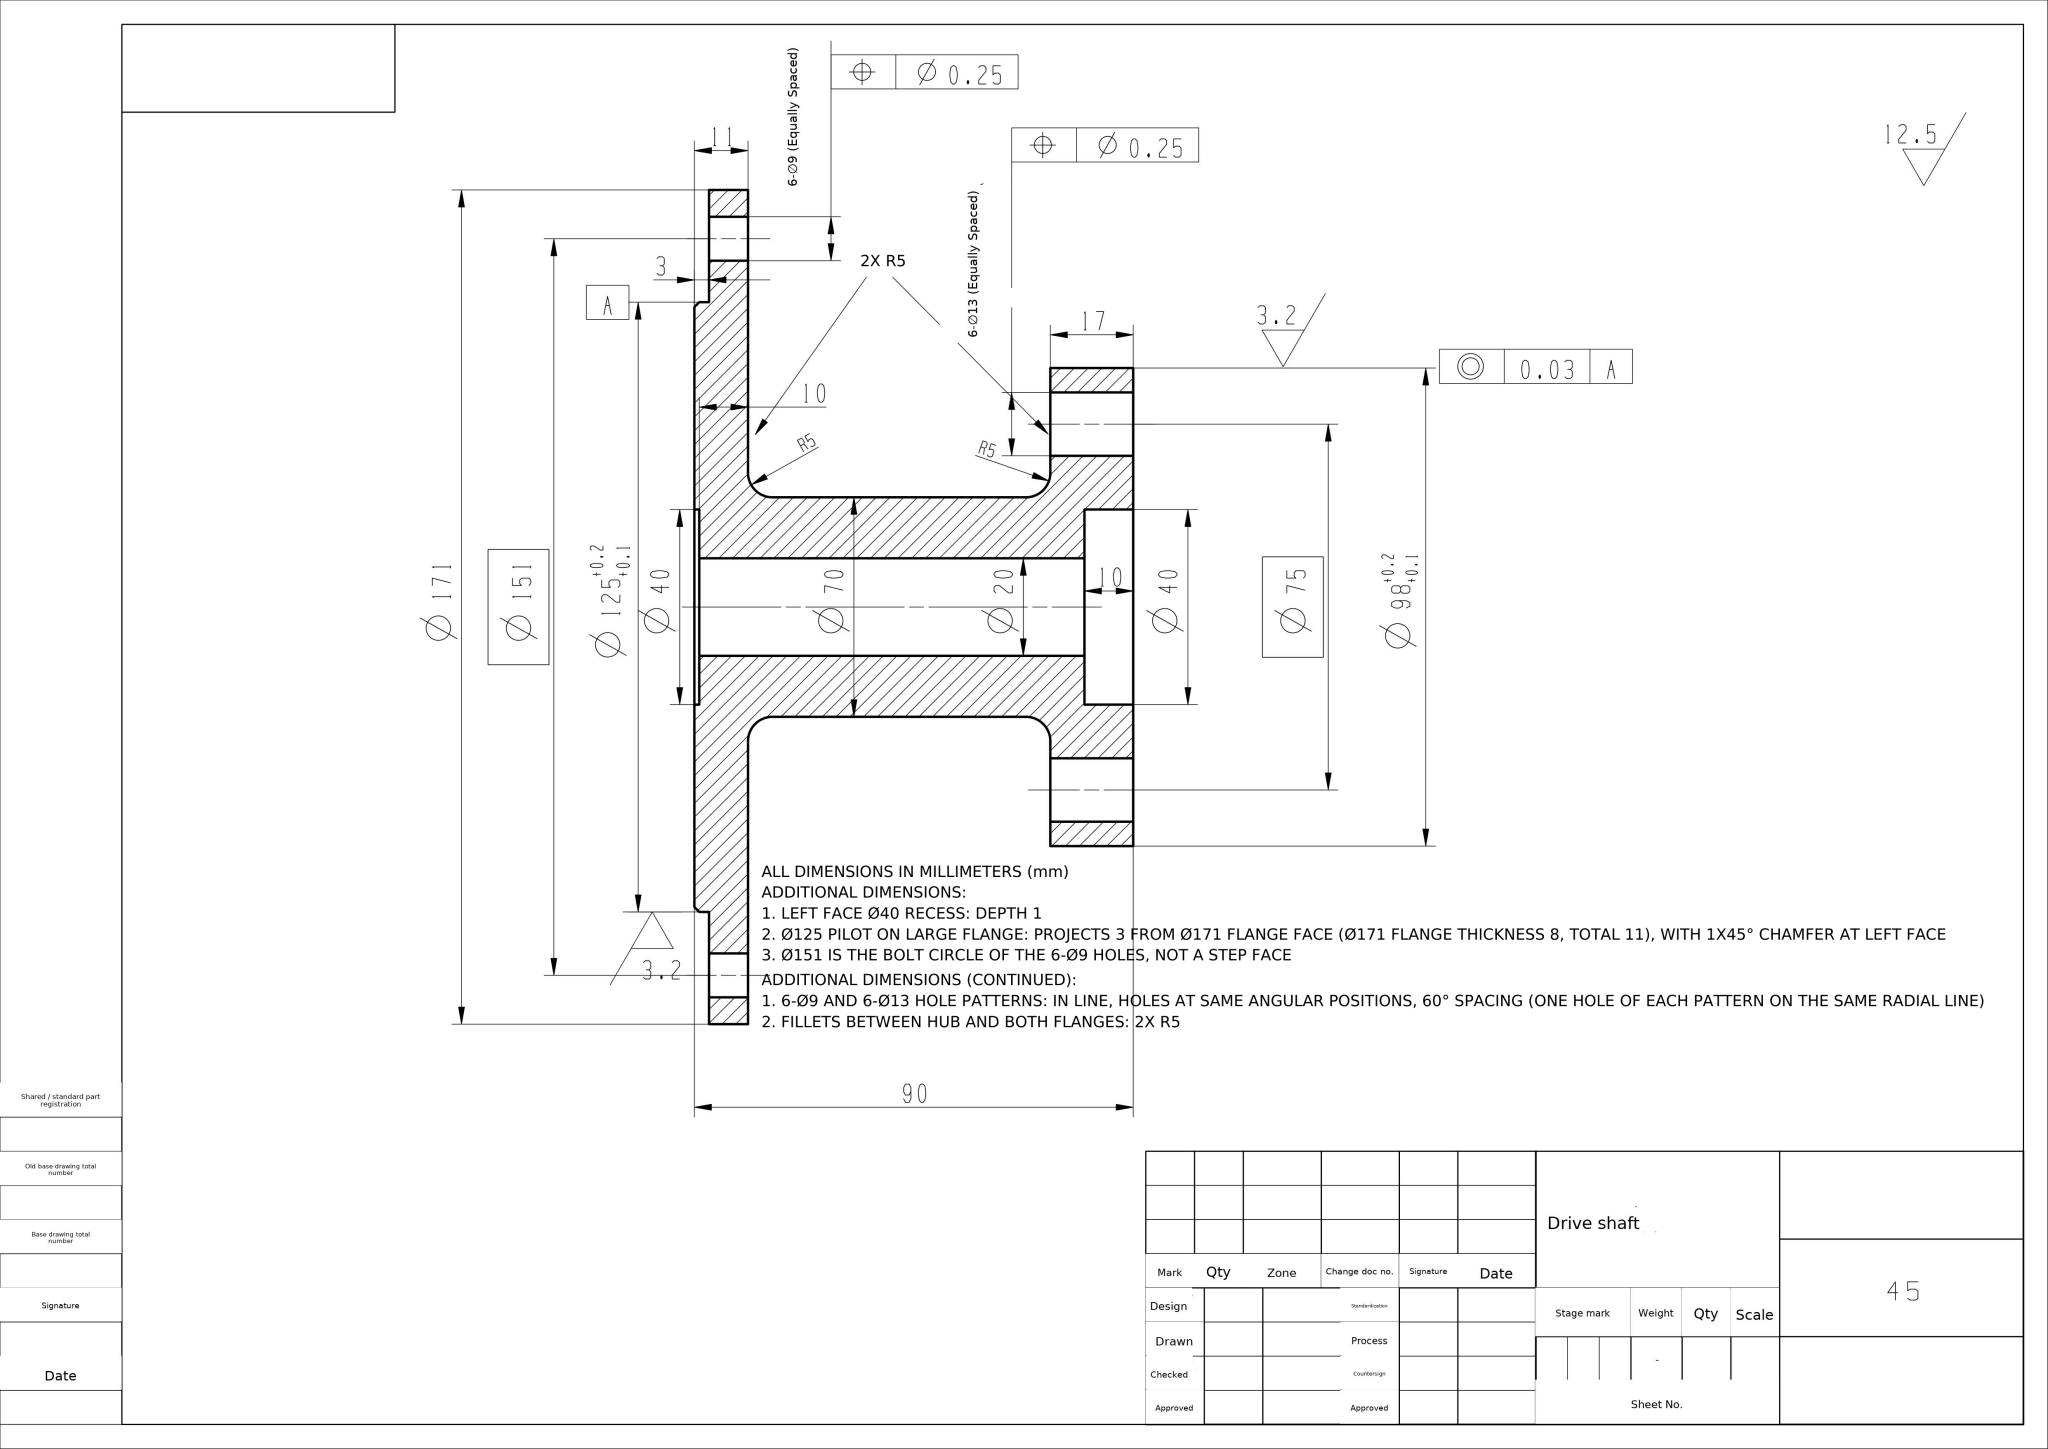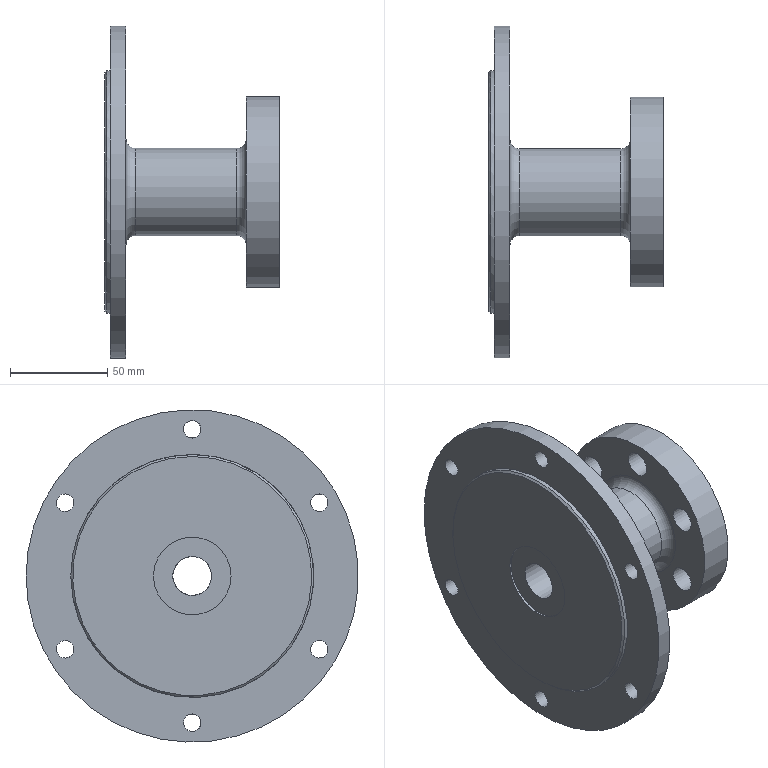Part | NX | mm | 1 solid | 29 faces | box 90 x 171 x 171 mm | volume 393542 mm3 | cylinder 19 | plane 7 | torus 2 | cone 1 | commonest cylinder face diameters 13 x6 9 x6 40 x2 45 x1 98 x1 171 x1 125 x1 20 x1
STEP:
#1=CARTESIAN_POINT('',(0.,0.,0.));
#2=DIRECTION('',(0.,0.,1.));
#3=DIRECTION('',(1.,0.,0.));
#4=AXIS2_PLACEMENT_3D('',#1,#2,#3);
#5=(LENGTH_UNIT()NAMED_UNIT(*)SI_UNIT(.MILLI.,.METRE.));
#6=UNCERTAINTY_MEASURE_WITH_UNIT(LENGTH_MEASURE(0.00002),#5,'','');
#7=(NAMED_UNIT(*)PLANE_ANGLE_UNIT()SI_UNIT($,.RADIAN.));
#8=PLANE_ANGLE_MEASURE_WITH_UNIT(PLANE_ANGLE_MEASURE(0.01745),#7);
#9=DIMENSIONAL_EXPONENTS(0.,0.,0.,0.,0.,0.,0.);
#10=(CONVERSION_BASED_UNIT('',#8)NAMED_UNIT(#9)PLANE_ANGLE_UNIT());
#11=(NAMED_UNIT(*)SI_UNIT($,.STERADIAN.)SOLID_ANGLE_UNIT());
#12=(GEOMETRIC_REPRESENTATION_CONTEXT(3)GLOBAL_UNCERTAINTY_ASSIGNED_CONTEXT((#6))GLOBAL_UNIT_ASSIGNED_CONTEXT((#5,#10,#11))REPRESENTATION_CONTEXT('',''));
#13=SHAPE_REPRESENTATION('',(#4),#12);
#14=CARTESIAN_POINT('',(-57.,0.,22.5));
#15=VERTEX_POINT('',#14);
#16=CARTESIAN_POINT('',(-57.,0.,0.));
#17=DIRECTION('',(1.,0.,0.));
#18=DIRECTION('',(0.,0.,1.));
#19=AXIS2_PLACEMENT_3D('',#16,#17,#18);
#20=CIRCLE('',#19,22.5);
#21=EDGE_CURVE('',#15,#15,#20,.T.);
#22=ORIENTED_EDGE('',*,*,#21,.T.);
#23=EDGE_LOOP('',(#22));
#24=FACE_BOUND('',#23,.T.);
#25=CARTESIAN_POINT('',(-5.,0.,-22.5));
#26=VERTEX_POINT('',#25);
#27=CARTESIAN_POINT('',(-5.,0.,0.));
#28=DIRECTION('',(-1.,0.,0.));
#29=DIRECTION('',(0.,0.,-1.));
#30=AXIS2_PLACEMENT_3D('',#27,#28,#29);
#31=CIRCLE('',#30,22.5);
#32=EDGE_CURVE('',#26,#26,#31,.T.);
#33=ORIENTED_EDGE('',*,*,#32,.T.);
#34=EDGE_LOOP('',(#33));
#35=FACE_BOUND('',#34,.T.);
#36=CARTESIAN_POINT('',(-62.,0.,0.));
#37=DIRECTION('',(1.,0.,0.));
#38=DIRECTION('',(0.,0.,-1.));
#39=AXIS2_PLACEMENT_3D('',#36,#37,#38);
#40=CYLINDRICAL_SURFACE('',#39,22.5);
#41=ADVANCED_FACE('',(#24,#35),#40,.T.);
#42=CARTESIAN_POINT('',(17.,0.,-20.));
#43=VERTEX_POINT('',#42);
#44=CARTESIAN_POINT('',(17.,0.,0.));
#45=DIRECTION('',(1.,0.,0.));
#46=DIRECTION('',(0.,0.,-1.));
#47=AXIS2_PLACEMENT_3D('',#44,#45,#46);
#48=CIRCLE('',#47,20.);
#49=EDGE_CURVE('',#43,#43,#48,.T.);
#50=ORIENTED_EDGE('',*,*,#49,.T.);
#51=EDGE_LOOP('',(#50));
#52=FACE_BOUND('',#51,.T.);
#53=CARTESIAN_POINT('',(7.,20.,-0.));
#54=VERTEX_POINT('',#53);
#55=CARTESIAN_POINT('',(7.,0.,0.));
#56=DIRECTION('',(-1.,0.,0.));
#57=DIRECTION('',(0.,1.,-0.));
#58=AXIS2_PLACEMENT_3D('',#55,#56,#57);
#59=CIRCLE('',#58,20.);
#60=EDGE_CURVE('',#54,#54,#59,.T.);
#61=ORIENTED_EDGE('',*,*,#60,.T.);
#62=EDGE_LOOP('',(#61));
#63=FACE_BOUND('',#62,.T.);
#64=CARTESIAN_POINT('',(20.,0.,0.));
#65=DIRECTION('',(-1.,0.,0.));
#66=DIRECTION('',(0.,0.,1.));
#67=AXIS2_PLACEMENT_3D('',#64,#65,#66);
#68=CYLINDRICAL_SURFACE('',#67,20.);
#69=ADVANCED_FACE('',(#52,#63),#68,.F.);
#70=CARTESIAN_POINT('',(17.,49.,-0.));
#71=VERTEX_POINT('',#70);
#72=CARTESIAN_POINT('',(17.,0.,0.));
#73=DIRECTION('',(1.,0.,0.));
#74=DIRECTION('',(0.,1.,-0.));
#75=AXIS2_PLACEMENT_3D('',#72,#73,#74);
#76=CIRCLE('',#75,49.);
#77=EDGE_CURVE('',#71,#71,#76,.T.);
#78=ORIENTED_EDGE('',*,*,#77,.F.);
#79=EDGE_LOOP('',(#78));
#80=FACE_BOUND('',#79,.T.);
#81=CARTESIAN_POINT('',(0.,49.,-0.));
#82=VERTEX_POINT('',#81);
#83=CARTESIAN_POINT('',(0.,0.,0.));
#84=DIRECTION('',(1.,0.,0.));
#85=DIRECTION('',(0.,1.,-0.));
#86=AXIS2_PLACEMENT_3D('',#83,#84,#85);
#87=CIRCLE('',#86,49.);
#88=EDGE_CURVE('',#82,#82,#87,.T.);
#89=ORIENTED_EDGE('',*,*,#88,.T.);
#90=EDGE_LOOP('',(#89));
#91=FACE_BOUND('',#90,.T.);
#92=CARTESIAN_POINT('',(17.,0.,0.));
#93=DIRECTION('',(-1.,0.,0.));
#94=DIRECTION('',(0.,0.,1.));
#95=AXIS2_PLACEMENT_3D('',#92,#93,#94);
#96=CYLINDRICAL_SURFACE('',#95,49.);
#97=ADVANCED_FACE('',(#80,#91),#96,.T.);
#98=CARTESIAN_POINT('',(17.,32.476,12.25));
#99=VERTEX_POINT('',#98);
#100=CARTESIAN_POINT('',(17.,32.476,18.75));
#101=DIRECTION('',(-1.,0.,0.));
#102=DIRECTION('',(0.,0.,-1.));
#103=AXIS2_PLACEMENT_3D('',#100,#101,#102);
#104=CIRCLE('',#103,6.5);
#105=EDGE_CURVE('',#99,#99,#104,.T.);
#106=ORIENTED_EDGE('',*,*,#105,.T.);
#107=EDGE_LOOP('',(#106));
#108=FACE_BOUND('',#107,.T.);
#109=CARTESIAN_POINT('',(17.,32.476,-25.25));
#110=VERTEX_POINT('',#109);
#111=CARTESIAN_POINT('',(17.,32.476,-18.75));
#112=DIRECTION('',(-1.,0.,0.));
#113=DIRECTION('',(0.,0.,-1.));
#114=AXIS2_PLACEMENT_3D('',#111,#112,#113);
#115=CIRCLE('',#114,6.5);
#116=EDGE_CURVE('',#110,#110,#115,.T.);
#117=ORIENTED_EDGE('',*,*,#116,.T.);
#118=EDGE_LOOP('',(#117));
#119=FACE_BOUND('',#118,.T.);
#120=CARTESIAN_POINT('',(17.,-0.,-44.));
#121=VERTEX_POINT('',#120);
#122=CARTESIAN_POINT('',(17.,-0.,-37.5));
#123=DIRECTION('',(-1.,0.,0.));
#124=DIRECTION('',(0.,0.,-1.));
#125=AXIS2_PLACEMENT_3D('',#122,#123,#124);
#126=CIRCLE('',#125,6.5);
#127=EDGE_CURVE('',#121,#121,#126,.T.);
#128=ORIENTED_EDGE('',*,*,#127,.T.);
#129=EDGE_LOOP('',(#128));
#130=FACE_BOUND('',#129,.T.);
#131=CARTESIAN_POINT('',(17.,-32.476,-25.25));
#132=VERTEX_POINT('',#131);
#133=CARTESIAN_POINT('',(17.,-32.476,-18.75));
#134=DIRECTION('',(-1.,0.,0.));
#135=DIRECTION('',(0.,0.,-1.));
#136=AXIS2_PLACEMENT_3D('',#133,#134,#135);
#137=CIRCLE('',#136,6.5);
#138=EDGE_CURVE('',#132,#132,#137,.T.);
#139=ORIENTED_EDGE('',*,*,#138,.T.);
#140=EDGE_LOOP('',(#139));
#141=FACE_BOUND('',#140,.T.);
#142=CARTESIAN_POINT('',(17.,-32.476,12.25));
#143=VERTEX_POINT('',#142);
#144=CARTESIAN_POINT('',(17.,-32.476,18.75));
#145=DIRECTION('',(-1.,0.,0.));
#146=DIRECTION('',(0.,0.,-1.));
#147=AXIS2_PLACEMENT_3D('',#144,#145,#146);
#148=CIRCLE('',#147,6.5);
#149=EDGE_CURVE('',#143,#143,#148,.T.);
#150=ORIENTED_EDGE('',*,*,#149,.T.);
#151=EDGE_LOOP('',(#150));
#152=FACE_BOUND('',#151,.T.);
#153=CARTESIAN_POINT('',(17.,-0.,31.));
#154=VERTEX_POINT('',#153);
#155=CARTESIAN_POINT('',(17.,-0.,37.5));
#156=DIRECTION('',(-1.,0.,0.));
#157=DIRECTION('',(0.,0.,-1.));
#158=AXIS2_PLACEMENT_3D('',#155,#156,#157);
#159=CIRCLE('',#158,6.5);
#160=EDGE_CURVE('',#154,#154,#159,.T.);
#161=ORIENTED_EDGE('',*,*,#160,.T.);
#162=EDGE_LOOP('',(#161));
#163=FACE_BOUND('',#162,.T.);
#164=ORIENTED_EDGE('',*,*,#49,.F.);
#165=EDGE_LOOP('',(#164));
#166=FACE_BOUND('',#165,.T.);
#167=ORIENTED_EDGE('',*,*,#77,.T.);
#168=EDGE_LOOP('',(#167));
#169=FACE_BOUND('',#168,.T.);
#170=CARTESIAN_POINT('',(17.,0.,0.));
#171=DIRECTION('',(1.,0.,0.));
#172=DIRECTION('',(0.,0.,-1.));
#173=AXIS2_PLACEMENT_3D('',#170,#171,#172);
#174=PLANE('',#173);
#175=ADVANCED_FACE('',(#108,#119,#130,#141,#152,#163,#166,#169),#174,.T.);
#176=CARTESIAN_POINT('',(0.,0.,-27.5));
#177=VERTEX_POINT('',#176);
#178=CARTESIAN_POINT('',(0.,0.,0.));
#179=DIRECTION('',(1.,0.,0.));
#180=DIRECTION('',(0.,0.,-1.));
#181=AXIS2_PLACEMENT_3D('',#178,#179,#180);
#182=CIRCLE('',#181,27.5);
#183=EDGE_CURVE('',#177,#177,#182,.T.);
#184=ORIENTED_EDGE('',*,*,#183,.T.);
#185=EDGE_LOOP('',(#184));
#186=FACE_BOUND('',#185,.T.);
#187=CARTESIAN_POINT('',(0.,35.726,13.121));
#188=VERTEX_POINT('',#187);
#189=CARTESIAN_POINT('',(0.,32.476,18.75));
#190=DIRECTION('',(1.,0.,0.));
#191=DIRECTION('',(0.,0.5,-0.866));
#192=AXIS2_PLACEMENT_3D('',#189,#190,#191);
#193=CIRCLE('',#192,6.5);
#194=EDGE_CURVE('',#188,#188,#193,.T.);
#195=ORIENTED_EDGE('',*,*,#194,.T.);
#196=EDGE_LOOP('',(#195));
#197=FACE_BOUND('',#196,.T.);
#198=CARTESIAN_POINT('',(0.,29.226,-24.379));
#199=VERTEX_POINT('',#198);
#200=CARTESIAN_POINT('',(0.,32.476,-18.75));
#201=DIRECTION('',(1.,0.,0.));
#202=DIRECTION('',(0.,-0.5,-0.866));
#203=AXIS2_PLACEMENT_3D('',#200,#201,#202);
#204=CIRCLE('',#203,6.5);
#205=EDGE_CURVE('',#199,#199,#204,.T.);
#206=ORIENTED_EDGE('',*,*,#205,.T.);
#207=EDGE_LOOP('',(#206));
#208=FACE_BOUND('',#207,.T.);
#209=CARTESIAN_POINT('',(0.,-6.5,-37.5));
#210=VERTEX_POINT('',#209);
#211=CARTESIAN_POINT('',(0.,-0.,-37.5));
#212=DIRECTION('',(1.,0.,0.));
#213=DIRECTION('',(0.,-1.,0.));
#214=AXIS2_PLACEMENT_3D('',#211,#212,#213);
#215=CIRCLE('',#214,6.5);
#216=EDGE_CURVE('',#210,#210,#215,.T.);
#217=ORIENTED_EDGE('',*,*,#216,.T.);
#218=EDGE_LOOP('',(#217));
#219=FACE_BOUND('',#218,.T.);
#220=CARTESIAN_POINT('',(0.,-35.726,-13.121));
#221=VERTEX_POINT('',#220);
#222=CARTESIAN_POINT('',(0.,-32.476,-18.75));
#223=DIRECTION('',(1.,0.,0.));
#224=DIRECTION('',(0.,-0.5,0.866));
#225=AXIS2_PLACEMENT_3D('',#222,#223,#224);
#226=CIRCLE('',#225,6.5);
#227=EDGE_CURVE('',#221,#221,#226,.T.);
#228=ORIENTED_EDGE('',*,*,#227,.T.);
#229=EDGE_LOOP('',(#228));
#230=FACE_BOUND('',#229,.T.);
#231=CARTESIAN_POINT('',(0.,-29.226,24.379));
#232=VERTEX_POINT('',#231);
#233=CARTESIAN_POINT('',(0.,-32.476,18.75));
#234=DIRECTION('',(1.,0.,0.));
#235=DIRECTION('',(0.,0.5,0.866));
#236=AXIS2_PLACEMENT_3D('',#233,#234,#235);
#237=CIRCLE('',#236,6.5);
#238=EDGE_CURVE('',#232,#232,#237,.T.);
#239=ORIENTED_EDGE('',*,*,#238,.T.);
#240=EDGE_LOOP('',(#239));
#241=FACE_BOUND('',#240,.T.);
#242=CARTESIAN_POINT('',(0.,6.5,37.5));
#243=VERTEX_POINT('',#242);
#244=CARTESIAN_POINT('',(0.,-0.,37.5));
#245=DIRECTION('',(1.,0.,0.));
#246=DIRECTION('',(0.,1.,0.));
#247=AXIS2_PLACEMENT_3D('',#244,#245,#246);
#248=CIRCLE('',#247,6.5);
#249=EDGE_CURVE('',#243,#243,#248,.T.);
#250=ORIENTED_EDGE('',*,*,#249,.T.);
#251=EDGE_LOOP('',(#250));
#252=FACE_BOUND('',#251,.T.);
#253=ORIENTED_EDGE('',*,*,#88,.F.);
#254=EDGE_LOOP('',(#253));
#255=FACE_BOUND('',#254,.T.);
#256=CARTESIAN_POINT('',(0.,0.,0.));
#257=DIRECTION('',(1.,0.,0.));
#258=DIRECTION('',(0.,0.,-1.));
#259=AXIS2_PLACEMENT_3D('',#256,#257,#258);
#260=PLANE('',#259);
#261=ADVANCED_FACE('',(#186,#197,#208,#219,#230,#241,#252,#255),#260,.F.);
#262=ORIENTED_EDGE('',*,*,#160,.F.);
#263=EDGE_LOOP('',(#262));
#264=FACE_BOUND('',#263,.T.);
#265=ORIENTED_EDGE('',*,*,#249,.F.);
#266=EDGE_LOOP('',(#265));
#267=FACE_BOUND('',#266,.T.);
#268=CARTESIAN_POINT('',(20.,-0.,37.5));
#269=DIRECTION('',(-1.,0.,0.));
#270=DIRECTION('',(0.,0.,1.));
#271=AXIS2_PLACEMENT_3D('',#268,#269,#270);
#272=CYLINDRICAL_SURFACE('',#271,6.5);
#273=ADVANCED_FACE('',(#264,#267),#272,.F.);
#274=ORIENTED_EDGE('',*,*,#149,.F.);
#275=EDGE_LOOP('',(#274));
#276=FACE_BOUND('',#275,.T.);
#277=ORIENTED_EDGE('',*,*,#238,.F.);
#278=EDGE_LOOP('',(#277));
#279=FACE_BOUND('',#278,.T.);
#280=CARTESIAN_POINT('',(20.,-32.476,18.75));
#281=DIRECTION('',(-1.,0.,0.));
#282=DIRECTION('',(0.,0.,1.));
#283=AXIS2_PLACEMENT_3D('',#280,#281,#282);
#284=CYLINDRICAL_SURFACE('',#283,6.5);
#285=ADVANCED_FACE('',(#276,#279),#284,.F.);
#286=ORIENTED_EDGE('',*,*,#138,.F.);
#287=EDGE_LOOP('',(#286));
#288=FACE_BOUND('',#287,.T.);
#289=ORIENTED_EDGE('',*,*,#227,.F.);
#290=EDGE_LOOP('',(#289));
#291=FACE_BOUND('',#290,.T.);
#292=CARTESIAN_POINT('',(20.,-32.476,-18.75));
#293=DIRECTION('',(-1.,0.,0.));
#294=DIRECTION('',(0.,0.,1.));
#295=AXIS2_PLACEMENT_3D('',#292,#293,#294);
#296=CYLINDRICAL_SURFACE('',#295,6.5);
#297=ADVANCED_FACE('',(#288,#291),#296,.F.);
#298=ORIENTED_EDGE('',*,*,#127,.F.);
#299=EDGE_LOOP('',(#298));
#300=FACE_BOUND('',#299,.T.);
#301=ORIENTED_EDGE('',*,*,#216,.F.);
#302=EDGE_LOOP('',(#301));
#303=FACE_BOUND('',#302,.T.);
#304=CARTESIAN_POINT('',(20.,-0.,-37.5));
#305=DIRECTION('',(-1.,0.,0.));
#306=DIRECTION('',(0.,0.,1.));
#307=AXIS2_PLACEMENT_3D('',#304,#305,#306);
#308=CYLINDRICAL_SURFACE('',#307,6.5);
#309=ADVANCED_FACE('',(#300,#303),#308,.F.);
#310=ORIENTED_EDGE('',*,*,#116,.F.);
#311=EDGE_LOOP('',(#310));
#312=FACE_BOUND('',#311,.T.);
#313=ORIENTED_EDGE('',*,*,#205,.F.);
#314=EDGE_LOOP('',(#313));
#315=FACE_BOUND('',#314,.T.);
#316=CARTESIAN_POINT('',(20.,32.476,-18.75));
#317=DIRECTION('',(-1.,0.,0.));
#318=DIRECTION('',(0.,0.,1.));
#319=AXIS2_PLACEMENT_3D('',#316,#317,#318);
#320=CYLINDRICAL_SURFACE('',#319,6.5);
#321=ADVANCED_FACE('',(#312,#315),#320,.F.);
#322=ORIENTED_EDGE('',*,*,#105,.F.);
#323=EDGE_LOOP('',(#322));
#324=FACE_BOUND('',#323,.T.);
#325=ORIENTED_EDGE('',*,*,#194,.F.);
#326=EDGE_LOOP('',(#325));
#327=FACE_BOUND('',#326,.T.);
#328=CARTESIAN_POINT('',(20.,32.476,18.75));
#329=DIRECTION('',(-1.,0.,0.));
#330=DIRECTION('',(0.,0.,1.));
#331=AXIS2_PLACEMENT_3D('',#328,#329,#330);
#332=CYLINDRICAL_SURFACE('',#331,6.5);
#333=ADVANCED_FACE('',(#324,#327),#332,.F.);
#334=CARTESIAN_POINT('',(7.,10.,-0.));
#335=VERTEX_POINT('',#334);
#336=CARTESIAN_POINT('',(7.,0.,0.));
#337=DIRECTION('',(1.,0.,0.));
#338=DIRECTION('',(0.,1.,-0.));
#339=AXIS2_PLACEMENT_3D('',#336,#337,#338);
#340=CIRCLE('',#339,10.);
#341=EDGE_CURVE('',#335,#335,#340,.T.);
#342=ORIENTED_EDGE('',*,*,#341,.F.);
#343=EDGE_LOOP('',(#342));
#344=FACE_BOUND('',#343,.T.);
#345=ORIENTED_EDGE('',*,*,#60,.F.);
#346=EDGE_LOOP('',(#345));
#347=FACE_BOUND('',#346,.T.);
#348=CARTESIAN_POINT('',(7.,0.,0.));
#349=DIRECTION('',(1.,0.,0.));
#350=DIRECTION('',(0.,0.,-1.));
#351=AXIS2_PLACEMENT_3D('',#348,#349,#350);
#352=PLANE('',#351);
#353=ADVANCED_FACE('',(#344,#347),#352,.T.);
#354=CARTESIAN_POINT('',(-62.,0.,27.5));
#355=VERTEX_POINT('',#354);
#356=CARTESIAN_POINT('',(-62.,0.,0.));
#357=DIRECTION('',(-1.,0.,0.));
#358=DIRECTION('',(0.,0.,1.));
#359=AXIS2_PLACEMENT_3D('',#356,#357,#358);
#360=CIRCLE('',#359,27.5);
#361=EDGE_CURVE('',#355,#355,#360,.T.);
#362=ORIENTED_EDGE('',*,*,#361,.T.);
#363=EDGE_LOOP('',(#362));
#364=FACE_BOUND('',#363,.T.);
#365=CARTESIAN_POINT('',(-62.,85.5,0.));
#366=VERTEX_POINT('',#365);
#367=CARTESIAN_POINT('',(-62.,0.,0.));
#368=DIRECTION('',(-1.,0.,0.));
#369=DIRECTION('',(0.,1.,0.));
#370=AXIS2_PLACEMENT_3D('',#367,#368,#369);
#371=CIRCLE('',#370,85.5);
#372=EDGE_CURVE('',#366,#366,#371,.T.);
#373=ORIENTED_EDGE('',*,*,#372,.F.);
#374=EDGE_LOOP('',(#373));
#375=FACE_BOUND('',#374,.T.);
#376=CARTESIAN_POINT('',(-62.,4.5,-75.5));
#377=VERTEX_POINT('',#376);
#378=CARTESIAN_POINT('',(-62.,0.,-75.5));
#379=DIRECTION('',(1.,0.,0.));
#380=DIRECTION('',(0.,1.,0.));
#381=AXIS2_PLACEMENT_3D('',#378,#379,#380);
#382=CIRCLE('',#381,4.5);
#383=EDGE_CURVE('',#377,#377,#382,.T.);
#384=ORIENTED_EDGE('',*,*,#383,.F.);
#385=EDGE_LOOP('',(#384));
#386=FACE_BOUND('',#385,.T.);
#387=CARTESIAN_POINT('',(-62.,67.635,-33.853));
#388=VERTEX_POINT('',#387);
#389=CARTESIAN_POINT('',(-62.,65.385,-37.75));
#390=DIRECTION('',(1.,0.,0.));
#391=DIRECTION('',(0.,0.5,0.866));
#392=AXIS2_PLACEMENT_3D('',#389,#390,#391);
#393=CIRCLE('',#392,4.5);
#394=EDGE_CURVE('',#388,#388,#393,.T.);
#395=ORIENTED_EDGE('',*,*,#394,.F.);
#396=EDGE_LOOP('',(#395));
#397=FACE_BOUND('',#396,.T.);
#398=CARTESIAN_POINT('',(-62.,63.135,41.647));
#399=VERTEX_POINT('',#398);
#400=CARTESIAN_POINT('',(-62.,65.385,37.75));
#401=DIRECTION('',(1.,0.,0.));
#402=DIRECTION('',(0.,-0.5,0.866));
#403=AXIS2_PLACEMENT_3D('',#400,#401,#402);
#404=CIRCLE('',#403,4.5);
#405=EDGE_CURVE('',#399,#399,#404,.T.);
#406=ORIENTED_EDGE('',*,*,#405,.F.);
#407=EDGE_LOOP('',(#406));
#408=FACE_BOUND('',#407,.T.);
#409=CARTESIAN_POINT('',(-62.,-4.5,75.5));
#410=VERTEX_POINT('',#409);
#411=CARTESIAN_POINT('',(-62.,0.,75.5));
#412=DIRECTION('',(1.,0.,0.));
#413=DIRECTION('',(0.,-1.,0.));
#414=AXIS2_PLACEMENT_3D('',#411,#412,#413);
#415=CIRCLE('',#414,4.5);
#416=EDGE_CURVE('',#410,#410,#415,.T.);
#417=ORIENTED_EDGE('',*,*,#416,.F.);
#418=EDGE_LOOP('',(#417));
#419=FACE_BOUND('',#418,.T.);
#420=CARTESIAN_POINT('',(-62.,-67.635,33.853));
#421=VERTEX_POINT('',#420);
#422=CARTESIAN_POINT('',(-62.,-65.385,37.75));
#423=DIRECTION('',(1.,0.,0.));
#424=DIRECTION('',(0.,-0.5,-0.866));
#425=AXIS2_PLACEMENT_3D('',#422,#423,#424);
#426=CIRCLE('',#425,4.5);
#427=EDGE_CURVE('',#421,#421,#426,.T.);
#428=ORIENTED_EDGE('',*,*,#427,.F.);
#429=EDGE_LOOP('',(#428));
#430=FACE_BOUND('',#429,.T.);
#431=CARTESIAN_POINT('',(-62.,-63.135,-41.647));
#432=VERTEX_POINT('',#431);
#433=CARTESIAN_POINT('',(-62.,-65.385,-37.75));
#434=DIRECTION('',(1.,0.,0.));
#435=DIRECTION('',(0.,0.5,-0.866));
#436=AXIS2_PLACEMENT_3D('',#433,#434,#435);
#437=CIRCLE('',#436,4.5);
#438=EDGE_CURVE('',#432,#432,#437,.T.);
#439=ORIENTED_EDGE('',*,*,#438,.F.);
#440=EDGE_LOOP('',(#439));
#441=FACE_BOUND('',#440,.T.);
#442=CARTESIAN_POINT('',(-62.,0.,0.));
#443=DIRECTION('',(-1.,0.,0.));
#444=DIRECTION('',(0.,0.,1.));
#445=AXIS2_PLACEMENT_3D('',#442,#443,#444);
#446=PLANE('',#445);
#447=ADVANCED_FACE('',(#364,#375,#386,#397,#408,#419,#430,#441),#446,.F.);
#448=ORIENTED_EDGE('',*,*,#372,.T.);
#449=EDGE_LOOP('',(#448));
#450=FACE_BOUND('',#449,.T.);
#451=CARTESIAN_POINT('',(-70.,85.5,0.));
#452=VERTEX_POINT('',#451);
#453=CARTESIAN_POINT('',(-70.,0.,0.));
#454=DIRECTION('',(-1.,0.,0.));
#455=DIRECTION('',(0.,1.,0.));
#456=AXIS2_PLACEMENT_3D('',#453,#454,#455);
#457=CIRCLE('',#456,85.5);
#458=EDGE_CURVE('',#452,#452,#457,.T.);
#459=ORIENTED_EDGE('',*,*,#458,.F.);
#460=EDGE_LOOP('',(#459));
#461=FACE_BOUND('',#460,.T.);
#462=CARTESIAN_POINT('',(-73.,0.,0.));
#463=DIRECTION('',(1.,0.,0.));
#464=DIRECTION('',(0.,0.,-1.));
#465=AXIS2_PLACEMENT_3D('',#462,#463,#464);
#466=CYLINDRICAL_SURFACE('',#465,85.5);
#467=ADVANCED_FACE('',(#450,#461),#466,.T.);
#468=CARTESIAN_POINT('',(-73.,0.,61.5));
#469=VERTEX_POINT('',#468);
#470=CARTESIAN_POINT('',(-73.,0.,0.));
#471=DIRECTION('',(-1.,0.,0.));
#472=DIRECTION('',(0.,0.,1.));
#473=AXIS2_PLACEMENT_3D('',#470,#471,#472);
#474=CIRCLE('',#473,61.5);
#475=EDGE_CURVE('',#469,#469,#474,.T.);
#476=ORIENTED_EDGE('',*,*,#475,.T.);
#477=EDGE_LOOP('',(#476));
#478=FACE_BOUND('',#477,.T.);
#479=CARTESIAN_POINT('',(-73.,20.,0.));
#480=VERTEX_POINT('',#479);
#481=CARTESIAN_POINT('',(-73.,0.,0.));
#482=DIRECTION('',(-1.,0.,0.));
#483=DIRECTION('',(0.,1.,0.));
#484=AXIS2_PLACEMENT_3D('',#481,#482,#483);
#485=CIRCLE('',#484,20.);
#486=EDGE_CURVE('',#480,#480,#485,.T.);
#487=ORIENTED_EDGE('',*,*,#486,.F.);
#488=EDGE_LOOP('',(#487));
#489=FACE_BOUND('',#488,.T.);
#490=CARTESIAN_POINT('',(-73.,0.,0.));
#491=DIRECTION('',(-1.,0.,0.));
#492=DIRECTION('',(0.,0.,1.));
#493=AXIS2_PLACEMENT_3D('',#490,#491,#492);
#494=PLANE('',#493);
#495=ADVANCED_FACE('',(#478,#489),#494,.T.);
#496=CARTESIAN_POINT('',(-72.,20.,-0.));
#497=VERTEX_POINT('',#496);
#498=CARTESIAN_POINT('',(-72.,0.,0.));
#499=DIRECTION('',(1.,0.,0.));
#500=DIRECTION('',(0.,1.,-0.));
#501=AXIS2_PLACEMENT_3D('',#498,#499,#500);
#502=CIRCLE('',#501,20.);
#503=EDGE_CURVE('',#497,#497,#502,.T.);
#504=ORIENTED_EDGE('',*,*,#503,.T.);
#505=EDGE_LOOP('',(#504));
#506=FACE_BOUND('',#505,.T.);
#507=ORIENTED_EDGE('',*,*,#486,.T.);
#508=EDGE_LOOP('',(#507));
#509=FACE_BOUND('',#508,.T.);
#510=CARTESIAN_POINT('',(-73.,0.,0.));
#511=DIRECTION('',(1.,0.,0.));
#512=DIRECTION('',(0.,0.,-1.));
#513=AXIS2_PLACEMENT_3D('',#510,#511,#512);
#514=CYLINDRICAL_SURFACE('',#513,20.);
#515=ADVANCED_FACE('',(#506,#509),#514,.F.);
#516=CARTESIAN_POINT('',(-72.,0.,62.5));
#517=VERTEX_POINT('',#516);
#518=CARTESIAN_POINT('',(-72.,0.,0.));
#519=DIRECTION('',(1.,0.,0.));
#520=DIRECTION('',(0.,0.,1.));
#521=AXIS2_PLACEMENT_3D('',#518,#519,#520);
#522=CIRCLE('',#521,62.5);
#523=EDGE_CURVE('',#517,#517,#522,.T.);
#524=ORIENTED_EDGE('',*,*,#523,.T.);
#525=EDGE_LOOP('',(#524));
#526=FACE_BOUND('',#525,.T.);
#527=CARTESIAN_POINT('',(-70.,62.5,0.));
#528=VERTEX_POINT('',#527);
#529=CARTESIAN_POINT('',(-70.,0.,0.));
#530=DIRECTION('',(-1.,0.,0.));
#531=DIRECTION('',(0.,1.,0.));
#532=AXIS2_PLACEMENT_3D('',#529,#530,#531);
#533=CIRCLE('',#532,62.5);
#534=EDGE_CURVE('',#528,#528,#533,.T.);
#535=ORIENTED_EDGE('',*,*,#534,.T.);
#536=EDGE_LOOP('',(#535));
#537=FACE_BOUND('',#536,.T.);
#538=CARTESIAN_POINT('',(-73.,0.,0.));
#539=DIRECTION('',(1.,0.,0.));
#540=DIRECTION('',(0.,0.,-1.));
#541=AXIS2_PLACEMENT_3D('',#538,#539,#540);
#542=CYLINDRICAL_SURFACE('',#541,62.5);
#543=ADVANCED_FACE('',(#526,#537),#542,.T.);
#544=CARTESIAN_POINT('',(-70.,-65.385,-33.25));
#545=VERTEX_POINT('',#544);
#546=CARTESIAN_POINT('',(-70.,-65.385,-37.75));
#547=DIRECTION('',(-1.,0.,0.));
#548=DIRECTION('',(0.,0.,1.));
#549=AXIS2_PLACEMENT_3D('',#546,#547,#548);
#550=CIRCLE('',#549,4.5);
#551=EDGE_CURVE('',#545,#545,#550,.T.);
#552=ORIENTED_EDGE('',*,*,#551,.F.);
#553=EDGE_LOOP('',(#552));
#554=FACE_BOUND('',#553,.T.);
#555=CARTESIAN_POINT('',(-70.,-65.385,42.25));
#556=VERTEX_POINT('',#555);
#557=CARTESIAN_POINT('',(-70.,-65.385,37.75));
#558=DIRECTION('',(-1.,0.,0.));
#559=DIRECTION('',(0.,0.,1.));
#560=AXIS2_PLACEMENT_3D('',#557,#558,#559);
#561=CIRCLE('',#560,4.5);
#562=EDGE_CURVE('',#556,#556,#561,.T.);
#563=ORIENTED_EDGE('',*,*,#562,.F.);
#564=EDGE_LOOP('',(#563));
#565=FACE_BOUND('',#564,.T.);
#566=CARTESIAN_POINT('',(-70.,0.,80.));
#567=VERTEX_POINT('',#566);
#568=CARTESIAN_POINT('',(-70.,0.,75.5));
#569=DIRECTION('',(-1.,0.,0.));
#570=DIRECTION('',(0.,0.,1.));
#571=AXIS2_PLACEMENT_3D('',#568,#569,#570);
#572=CIRCLE('',#571,4.5);
#573=EDGE_CURVE('',#567,#567,#572,.T.);
#574=ORIENTED_EDGE('',*,*,#573,.F.);
#575=EDGE_LOOP('',(#574));
#576=FACE_BOUND('',#575,.T.);
#577=CARTESIAN_POINT('',(-70.,65.385,42.25));
#578=VERTEX_POINT('',#577);
#579=CARTESIAN_POINT('',(-70.,65.385,37.75));
#580=DIRECTION('',(-1.,0.,0.));
#581=DIRECTION('',(0.,0.,1.));
#582=AXIS2_PLACEMENT_3D('',#579,#580,#581);
#583=CIRCLE('',#582,4.5);
#584=EDGE_CURVE('',#578,#578,#583,.T.);
#585=ORIENTED_EDGE('',*,*,#584,.F.);
#586=EDGE_LOOP('',(#585));
#587=FACE_BOUND('',#586,.T.);
#588=CARTESIAN_POINT('',(-70.,65.385,-33.25));
#589=VERTEX_POINT('',#588);
#590=CARTESIAN_POINT('',(-70.,65.385,-37.75));
#591=DIRECTION('',(-1.,0.,0.));
#592=DIRECTION('',(0.,0.,1.));
#593=AXIS2_PLACEMENT_3D('',#590,#591,#592);
#594=CIRCLE('',#593,4.5);
#595=EDGE_CURVE('',#589,#589,#594,.T.);
#596=ORIENTED_EDGE('',*,*,#595,.F.);
#597=EDGE_LOOP('',(#596));
#598=FACE_BOUND('',#597,.T.);
#599=CARTESIAN_POINT('',(-70.,0.,-71.));
#600=VERTEX_POINT('',#599);
#601=CARTESIAN_POINT('',(-70.,0.,-75.5));
#602=DIRECTION('',(-1.,0.,0.));
#603=DIRECTION('',(0.,0.,1.));
#604=AXIS2_PLACEMENT_3D('',#601,#602,#603);
#605=CIRCLE('',#604,4.5);
#606=EDGE_CURVE('',#600,#600,#605,.T.);
#607=ORIENTED_EDGE('',*,*,#606,.F.);
#608=EDGE_LOOP('',(#607));
#609=FACE_BOUND('',#608,.T.);
#610=ORIENTED_EDGE('',*,*,#458,.T.);
#611=EDGE_LOOP('',(#610));
#612=FACE_BOUND('',#611,.T.);
#613=ORIENTED_EDGE('',*,*,#534,.F.);
#614=EDGE_LOOP('',(#613));
#615=FACE_BOUND('',#614,.T.);
#616=CARTESIAN_POINT('',(-70.,0.,0.));
#617=DIRECTION('',(-1.,0.,0.));
#618=DIRECTION('',(0.,0.,1.));
#619=AXIS2_PLACEMENT_3D('',#616,#617,#618);
#620=PLANE('',#619);
#621=ADVANCED_FACE('',(#554,#565,#576,#587,#598,#609,#612,#615),#620,.T.);
#622=ORIENTED_EDGE('',*,*,#475,.F.);
#623=EDGE_LOOP('',(#622));
#624=FACE_BOUND('',#623,.T.);
#625=ORIENTED_EDGE('',*,*,#523,.F.);
#626=EDGE_LOOP('',(#625));
#627=FACE_BOUND('',#626,.T.);
#628=CARTESIAN_POINT('',(-72.,0.,0.));
#629=DIRECTION('',(1.,0.,0.));
#630=DIRECTION('',(0.,0.,-1.));
#631=AXIS2_PLACEMENT_3D('',#628,#629,#630);
#632=CONICAL_SURFACE('',#631,62.5,45.);
#633=ADVANCED_FACE('',(#624,#627),#632,.T.);
#634=ORIENTED_EDGE('',*,*,#606,.T.);
#635=EDGE_LOOP('',(#634));
#636=FACE_BOUND('',#635,.T.);
#637=ORIENTED_EDGE('',*,*,#383,.T.);
#638=EDGE_LOOP('',(#637));
#639=FACE_BOUND('',#638,.T.);
#640=CARTESIAN_POINT('',(-82.,0.,-75.5));
#641=DIRECTION('',(1.,0.,0.));
#642=DIRECTION('',(0.,0.,-1.));
#643=AXIS2_PLACEMENT_3D('',#640,#641,#642);
#644=CYLINDRICAL_SURFACE('',#643,4.5);
#645=ADVANCED_FACE('',(#636,#639),#644,.F.);
#646=ORIENTED_EDGE('',*,*,#595,.T.);
#647=EDGE_LOOP('',(#646));
#648=FACE_BOUND('',#647,.T.);
#649=ORIENTED_EDGE('',*,*,#394,.T.);
#650=EDGE_LOOP('',(#649));
#651=FACE_BOUND('',#650,.T.);
#652=CARTESIAN_POINT('',(-82.,65.385,-37.75));
#653=DIRECTION('',(1.,0.,0.));
#654=DIRECTION('',(0.,0.,-1.));
#655=AXIS2_PLACEMENT_3D('',#652,#653,#654);
#656=CYLINDRICAL_SURFACE('',#655,4.5);
#657=ADVANCED_FACE('',(#648,#651),#656,.F.);
#658=ORIENTED_EDGE('',*,*,#584,.T.);
#659=EDGE_LOOP('',(#658));
#660=FACE_BOUND('',#659,.T.);
#661=ORIENTED_EDGE('',*,*,#405,.T.);
#662=EDGE_LOOP('',(#661));
#663=FACE_BOUND('',#662,.T.);
#664=CARTESIAN_POINT('',(-82.,65.385,37.75));
#665=DIRECTION('',(1.,0.,0.));
#666=DIRECTION('',(0.,0.,-1.));
#667=AXIS2_PLACEMENT_3D('',#664,#665,#666);
#668=CYLINDRICAL_SURFACE('',#667,4.5);
#669=ADVANCED_FACE('',(#660,#663),#668,.F.);
#670=ORIENTED_EDGE('',*,*,#573,.T.);
#671=EDGE_LOOP('',(#670));
#672=FACE_BOUND('',#671,.T.);
#673=ORIENTED_EDGE('',*,*,#416,.T.);
#674=EDGE_LOOP('',(#673));
#675=FACE_BOUND('',#674,.T.);
#676=CARTESIAN_POINT('',(-82.,0.,75.5));
#677=DIRECTION('',(1.,0.,0.));
#678=DIRECTION('',(0.,0.,-1.));
#679=AXIS2_PLACEMENT_3D('',#676,#677,#678);
#680=CYLINDRICAL_SURFACE('',#679,4.5);
#681=ADVANCED_FACE('',(#672,#675),#680,.F.);
#682=ORIENTED_EDGE('',*,*,#562,.T.);
#683=EDGE_LOOP('',(#682));
#684=FACE_BOUND('',#683,.T.);
#685=ORIENTED_EDGE('',*,*,#427,.T.);
#686=EDGE_LOOP('',(#685));
#687=FACE_BOUND('',#686,.T.);
#688=CARTESIAN_POINT('',(-82.,-65.385,37.75));
#689=DIRECTION('',(1.,0.,0.));
#690=DIRECTION('',(0.,0.,-1.));
#691=AXIS2_PLACEMENT_3D('',#688,#689,#690);
#692=CYLINDRICAL_SURFACE('',#691,4.5);
#693=ADVANCED_FACE('',(#684,#687),#692,.F.);
#694=ORIENTED_EDGE('',*,*,#551,.T.);
#695=EDGE_LOOP('',(#694));
#696=FACE_BOUND('',#695,.T.);
#697=ORIENTED_EDGE('',*,*,#438,.T.);
#698=EDGE_LOOP('',(#697));
#699=FACE_BOUND('',#698,.T.);
#700=CARTESIAN_POINT('',(-82.,-65.385,-37.75));
#701=DIRECTION('',(1.,0.,0.));
#702=DIRECTION('',(0.,0.,-1.));
#703=AXIS2_PLACEMENT_3D('',#700,#701,#702);
#704=CYLINDRICAL_SURFACE('',#703,4.5);
#705=ADVANCED_FACE('',(#696,#699),#704,.F.);
#706=CARTESIAN_POINT('',(-72.,0.,-10.));
#707=VERTEX_POINT('',#706);
#708=CARTESIAN_POINT('',(-72.,0.,0.));
#709=DIRECTION('',(1.,0.,0.));
#710=DIRECTION('',(0.,0.,-1.));
#711=AXIS2_PLACEMENT_3D('',#708,#709,#710);
#712=CIRCLE('',#711,10.);
#713=EDGE_CURVE('',#707,#707,#712,.T.);
#714=ORIENTED_EDGE('',*,*,#713,.T.);
#715=EDGE_LOOP('',(#714));
#716=FACE_BOUND('',#715,.T.);
#717=ORIENTED_EDGE('',*,*,#503,.F.);
#718=EDGE_LOOP('',(#717));
#719=FACE_BOUND('',#718,.T.);
#720=CARTESIAN_POINT('',(-72.,0.,0.));
#721=DIRECTION('',(1.,0.,0.));
#722=DIRECTION('',(0.,0.,-1.));
#723=AXIS2_PLACEMENT_3D('',#720,#721,#722);
#724=PLANE('',#723);
#725=ADVANCED_FACE('',(#716,#719),#724,.F.);
#726=ORIENTED_EDGE('',*,*,#21,.F.);
#727=EDGE_LOOP('',(#726));
#728=FACE_BOUND('',#727,.T.);
#729=ORIENTED_EDGE('',*,*,#361,.F.);
#730=EDGE_LOOP('',(#729));
#731=FACE_BOUND('',#730,.T.);
#732=CARTESIAN_POINT('',(-57.,0.,0.));
#733=DIRECTION('',(-1.,0.,0.));
#734=DIRECTION('',(0.,0.,1.));
#735=AXIS2_PLACEMENT_3D('',#732,#733,#734);
#736=TOROIDAL_SURFACE('',#735,27.5,5.);
#737=ADVANCED_FACE('',(#728,#731),#736,.F.);
#738=ORIENTED_EDGE('',*,*,#183,.F.);
#739=EDGE_LOOP('',(#738));
#740=FACE_BOUND('',#739,.T.);
#741=ORIENTED_EDGE('',*,*,#32,.F.);
#742=EDGE_LOOP('',(#741));
#743=FACE_BOUND('',#742,.T.);
#744=CARTESIAN_POINT('',(-5.,0.,0.));
#745=DIRECTION('',(1.,0.,0.));
#746=DIRECTION('',(0.,0.,-1.));
#747=AXIS2_PLACEMENT_3D('',#744,#745,#746);
#748=TOROIDAL_SURFACE('',#747,27.5,5.);
#749=ADVANCED_FACE('',(#740,#743),#748,.F.);
#750=ORIENTED_EDGE('',*,*,#341,.T.);
#751=EDGE_LOOP('',(#750));
#752=FACE_BOUND('',#751,.T.);
#753=ORIENTED_EDGE('',*,*,#713,.F.);
#754=EDGE_LOOP('',(#753));
#755=FACE_BOUND('',#754,.T.);
#756=CARTESIAN_POINT('',(-54993.,0.,0.));
#757=DIRECTION('',(1.,0.,0.));
#758=DIRECTION('',(0.,0.,-1.));
#759=AXIS2_PLACEMENT_3D('',#756,#757,#758);
#760=CYLINDRICAL_SURFACE('',#759,10.);
#761=ADVANCED_FACE('',(#752,#755),#760,.F.);
#762=CLOSED_SHELL('',(#41,#69,#97,#175,#261,#273,#285,#297,#309,#321,#333,#353,#447,#467,#495,#515,#543,#621,#633,#645,#657,#669,#681,#693,#705,#725,#737,#749,#761));
#763=MANIFOLD_SOLID_BREP('',#762);
#764=ADVANCED_BREP_SHAPE_REPRESENTATION('',(#763),#12);
#765=SHAPE_REPRESENTATION_RELATIONSHIP('','',#13,#764);
#766=PRESENTATION_LAYER_ASSIGNMENT('','',(#763));
#767=COLOUR_RGB('',1.,0.6,0.);
#768=FILL_AREA_STYLE_COLOUR('',#767);
#769=FILL_AREA_STYLE('',(#768));
#770=SURFACE_STYLE_FILL_AREA(#769);
#771=SURFACE_SIDE_STYLE('',(#770));
#772=SURFACE_STYLE_USAGE(.BOTH.,#771);
#773=PRESENTATION_STYLE_ASSIGNMENT((#772));
#774=STYLED_ITEM('',(#773),#763);
#775=MECHANICAL_DESIGN_GEOMETRIC_PRESENTATION_REPRESENTATION('',(#774),#12);